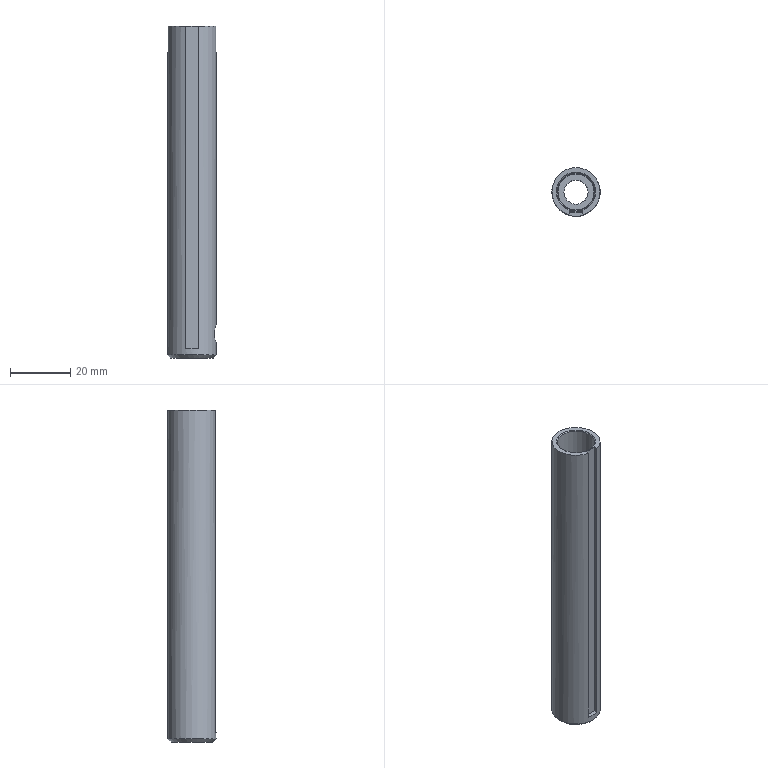Component | NX | SLEEVE | 1 solid | 15 faces | volume 11929 mm3 | plane 8 | cylinder 5 | cone 2 | commonest cylinder face diameters 16 x1 8 x1 12 x1 6.144 x1 12.427 x1